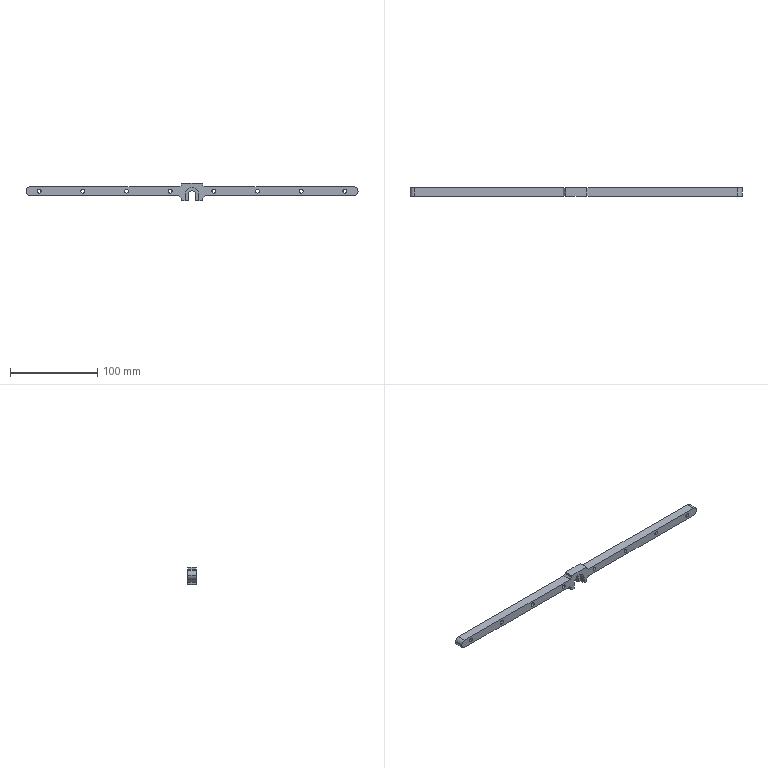Component | SolidWorks | 002MaterialPickingModuleB-1_004SidePlugModuleB-1_J-025-2 | 1 solid | 74 faces | volume 36274 mm3 | cylinder 40 | plane 34 | commonest cylinder face diameters 8 x16 4.5 x16 10 x4 9 x2 16 x2 | material 45